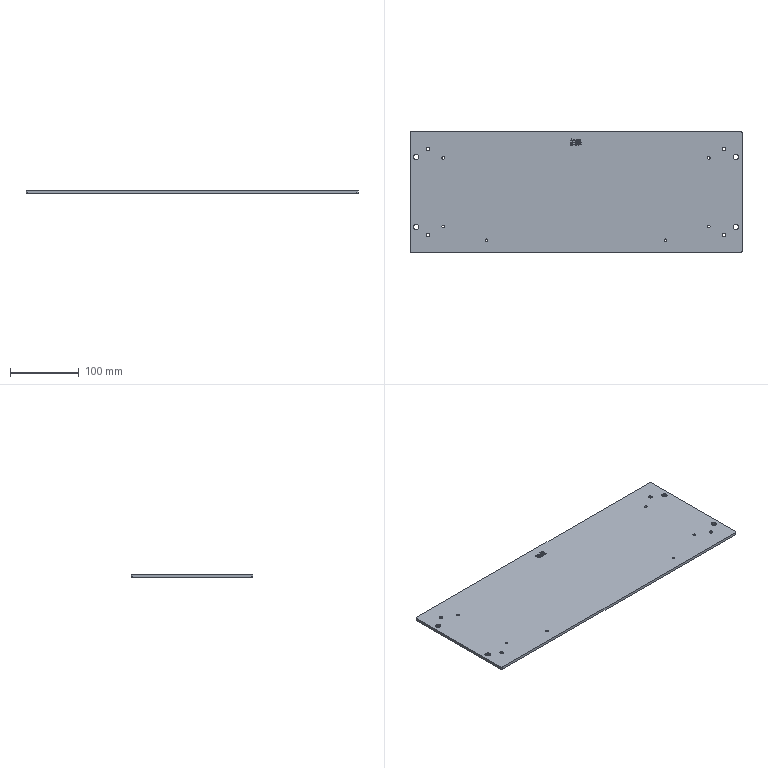CAM job | Mastercam | mm | 7 operations | part box 482.6 x 177 x 4
1. Contour (Ramp) | 9 - 10 平铣刀
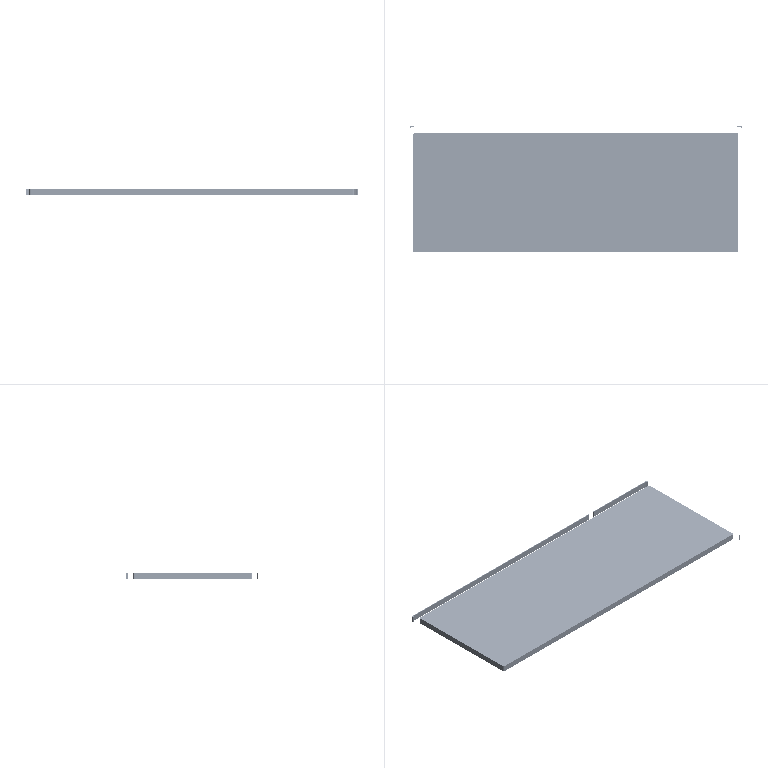2. Contour (2D) | 10 - 10 平铣刀
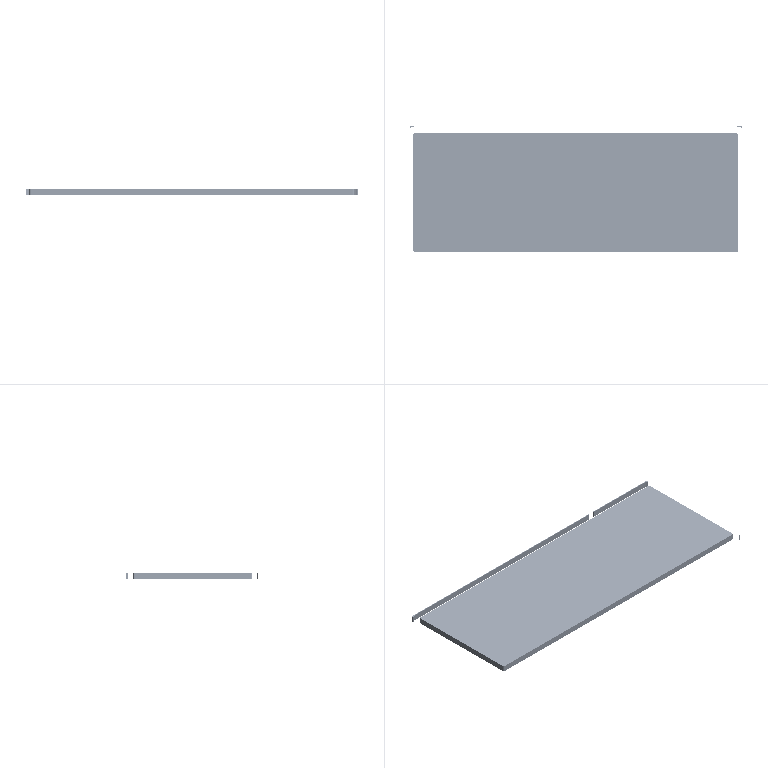3. Contour (Ramp) | 4 - 4 平铣刀
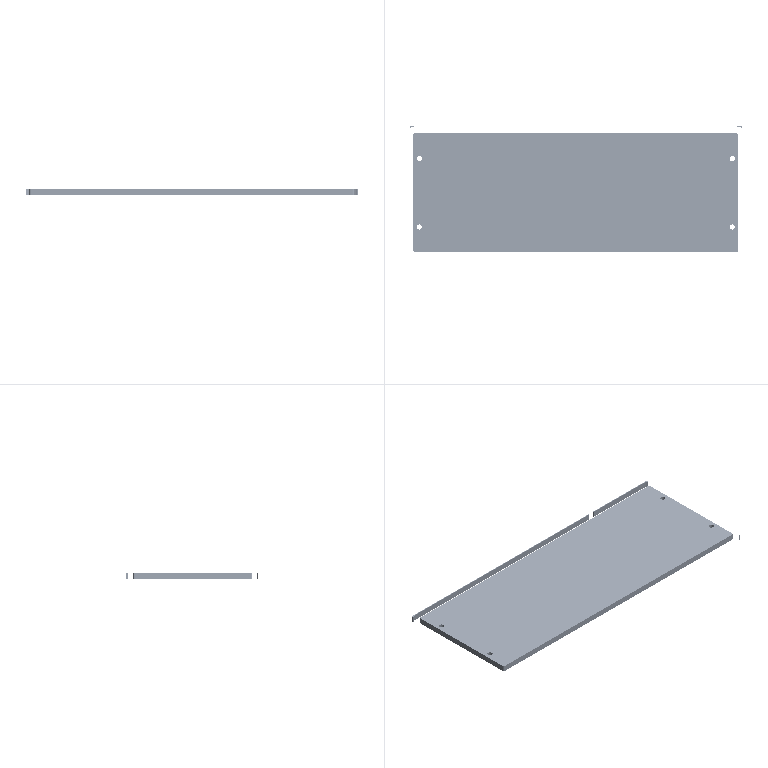4. 3D High Speed (Waterline) | 14 - 4 圆鼻铣刀
5. Contour (2D) | 3 - 3 平铣刀
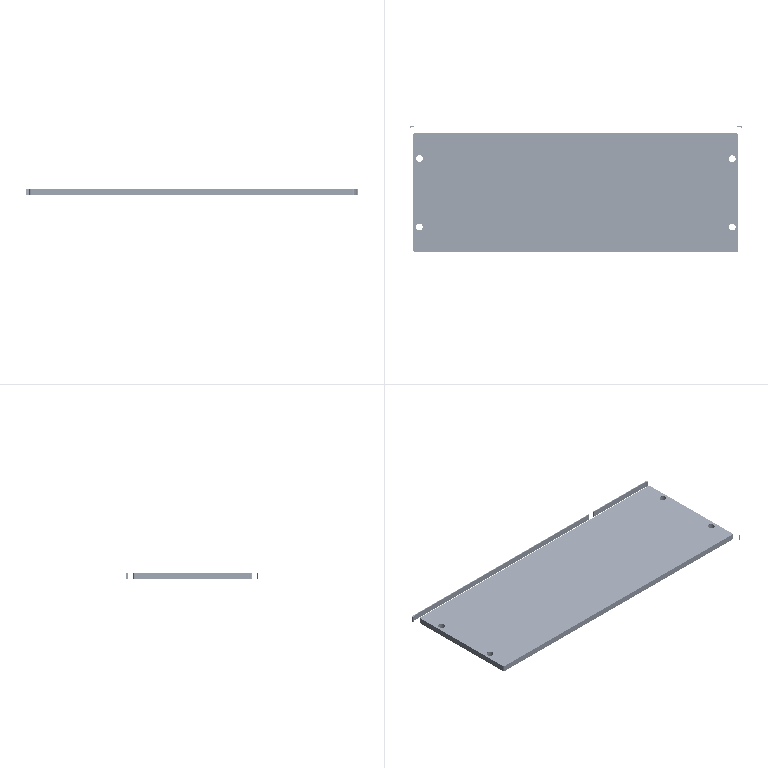6. Drill/Counterbore | 5 - 4 倒角刀
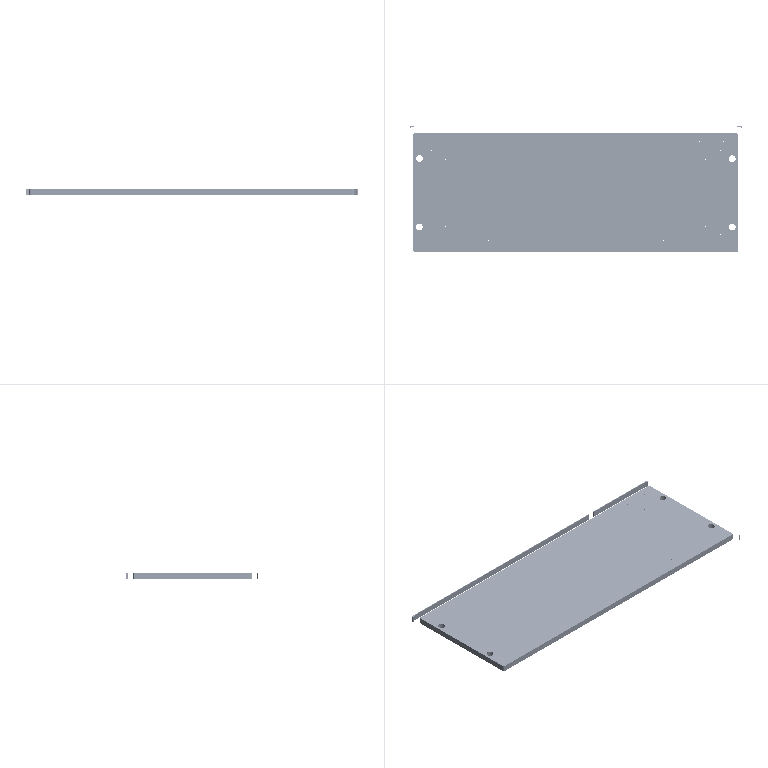7. Contour (2D chamfer) | 5 - 4 倒角刀